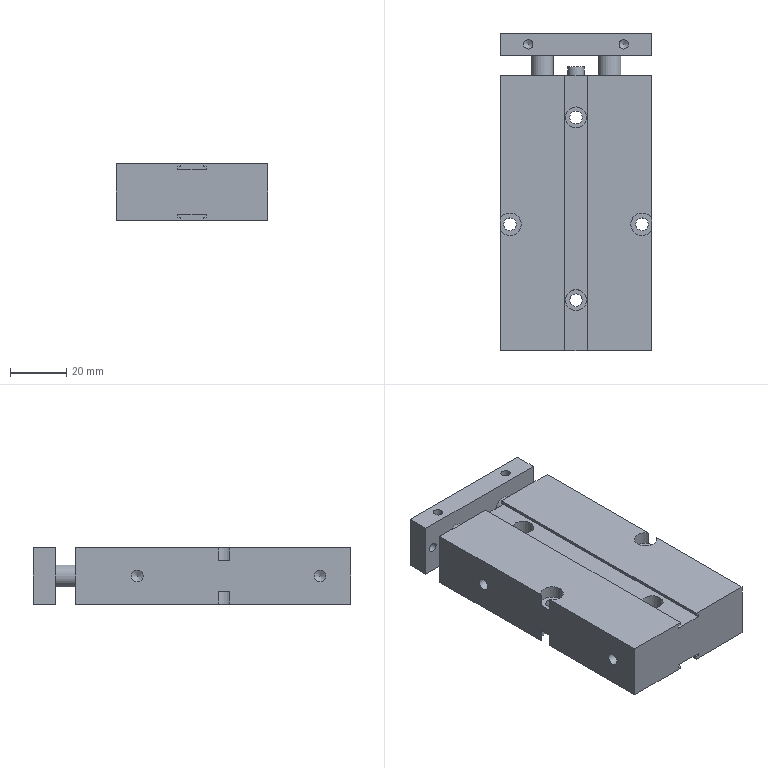Component | NX | DUAL_AXIS_CYLINDER | 5 solids | 81 faces | volume 107716 mm3 | plane 44 | cylinder 29 | cone 8 | commonest cylinder face diameters 8 x8 3.3 x6 4.5 x4 7.5 x4 4.2 x4 10 x2 6 x1